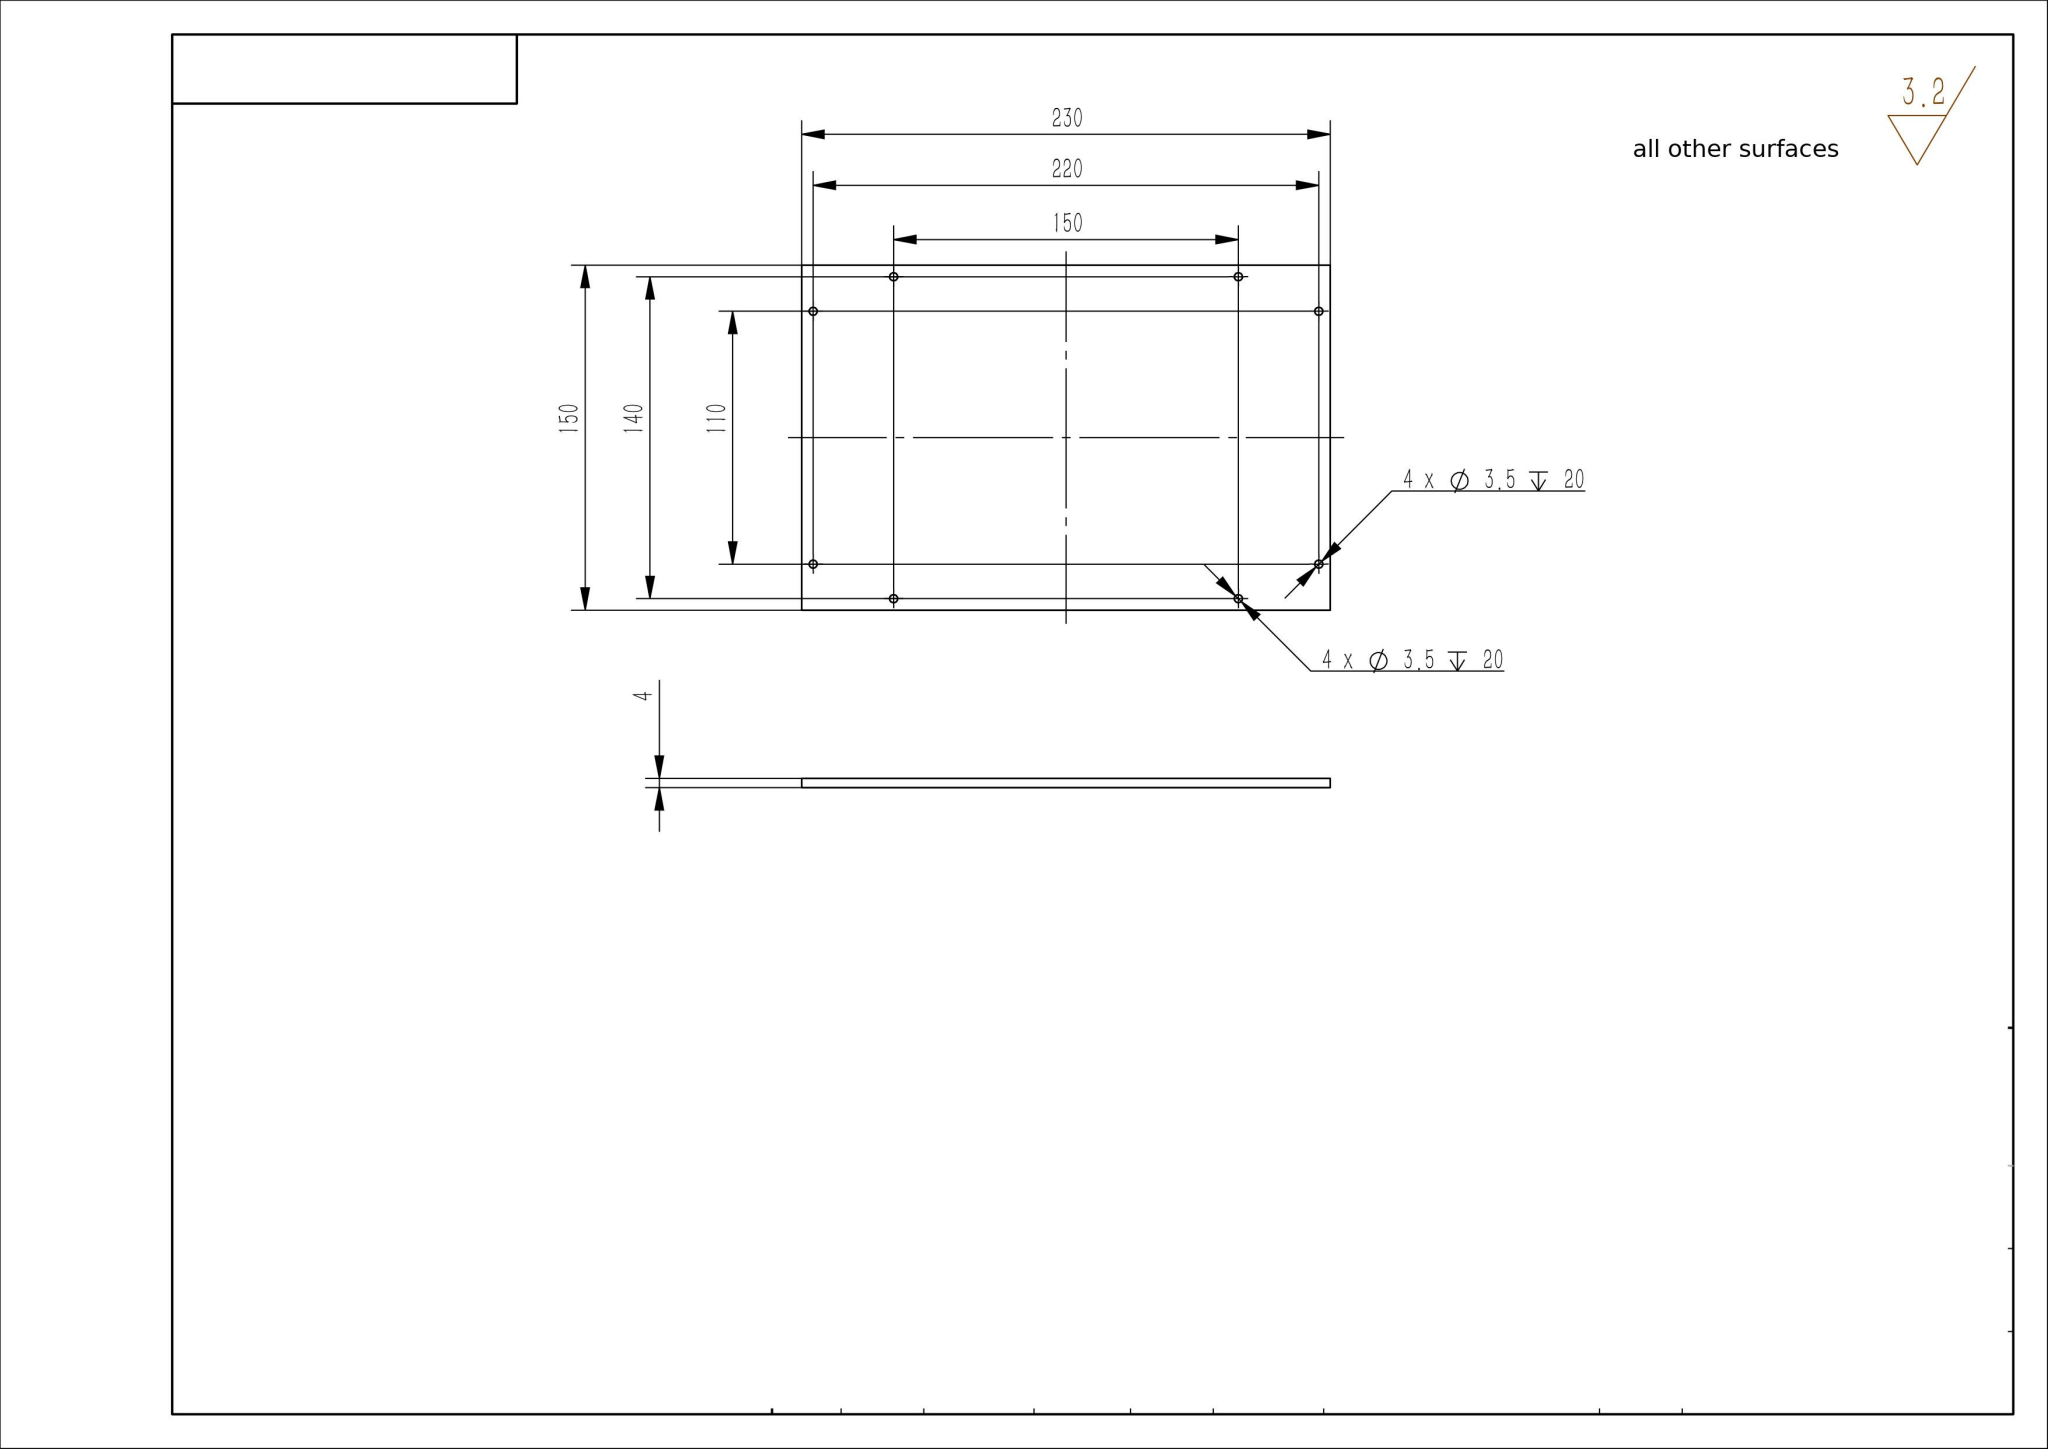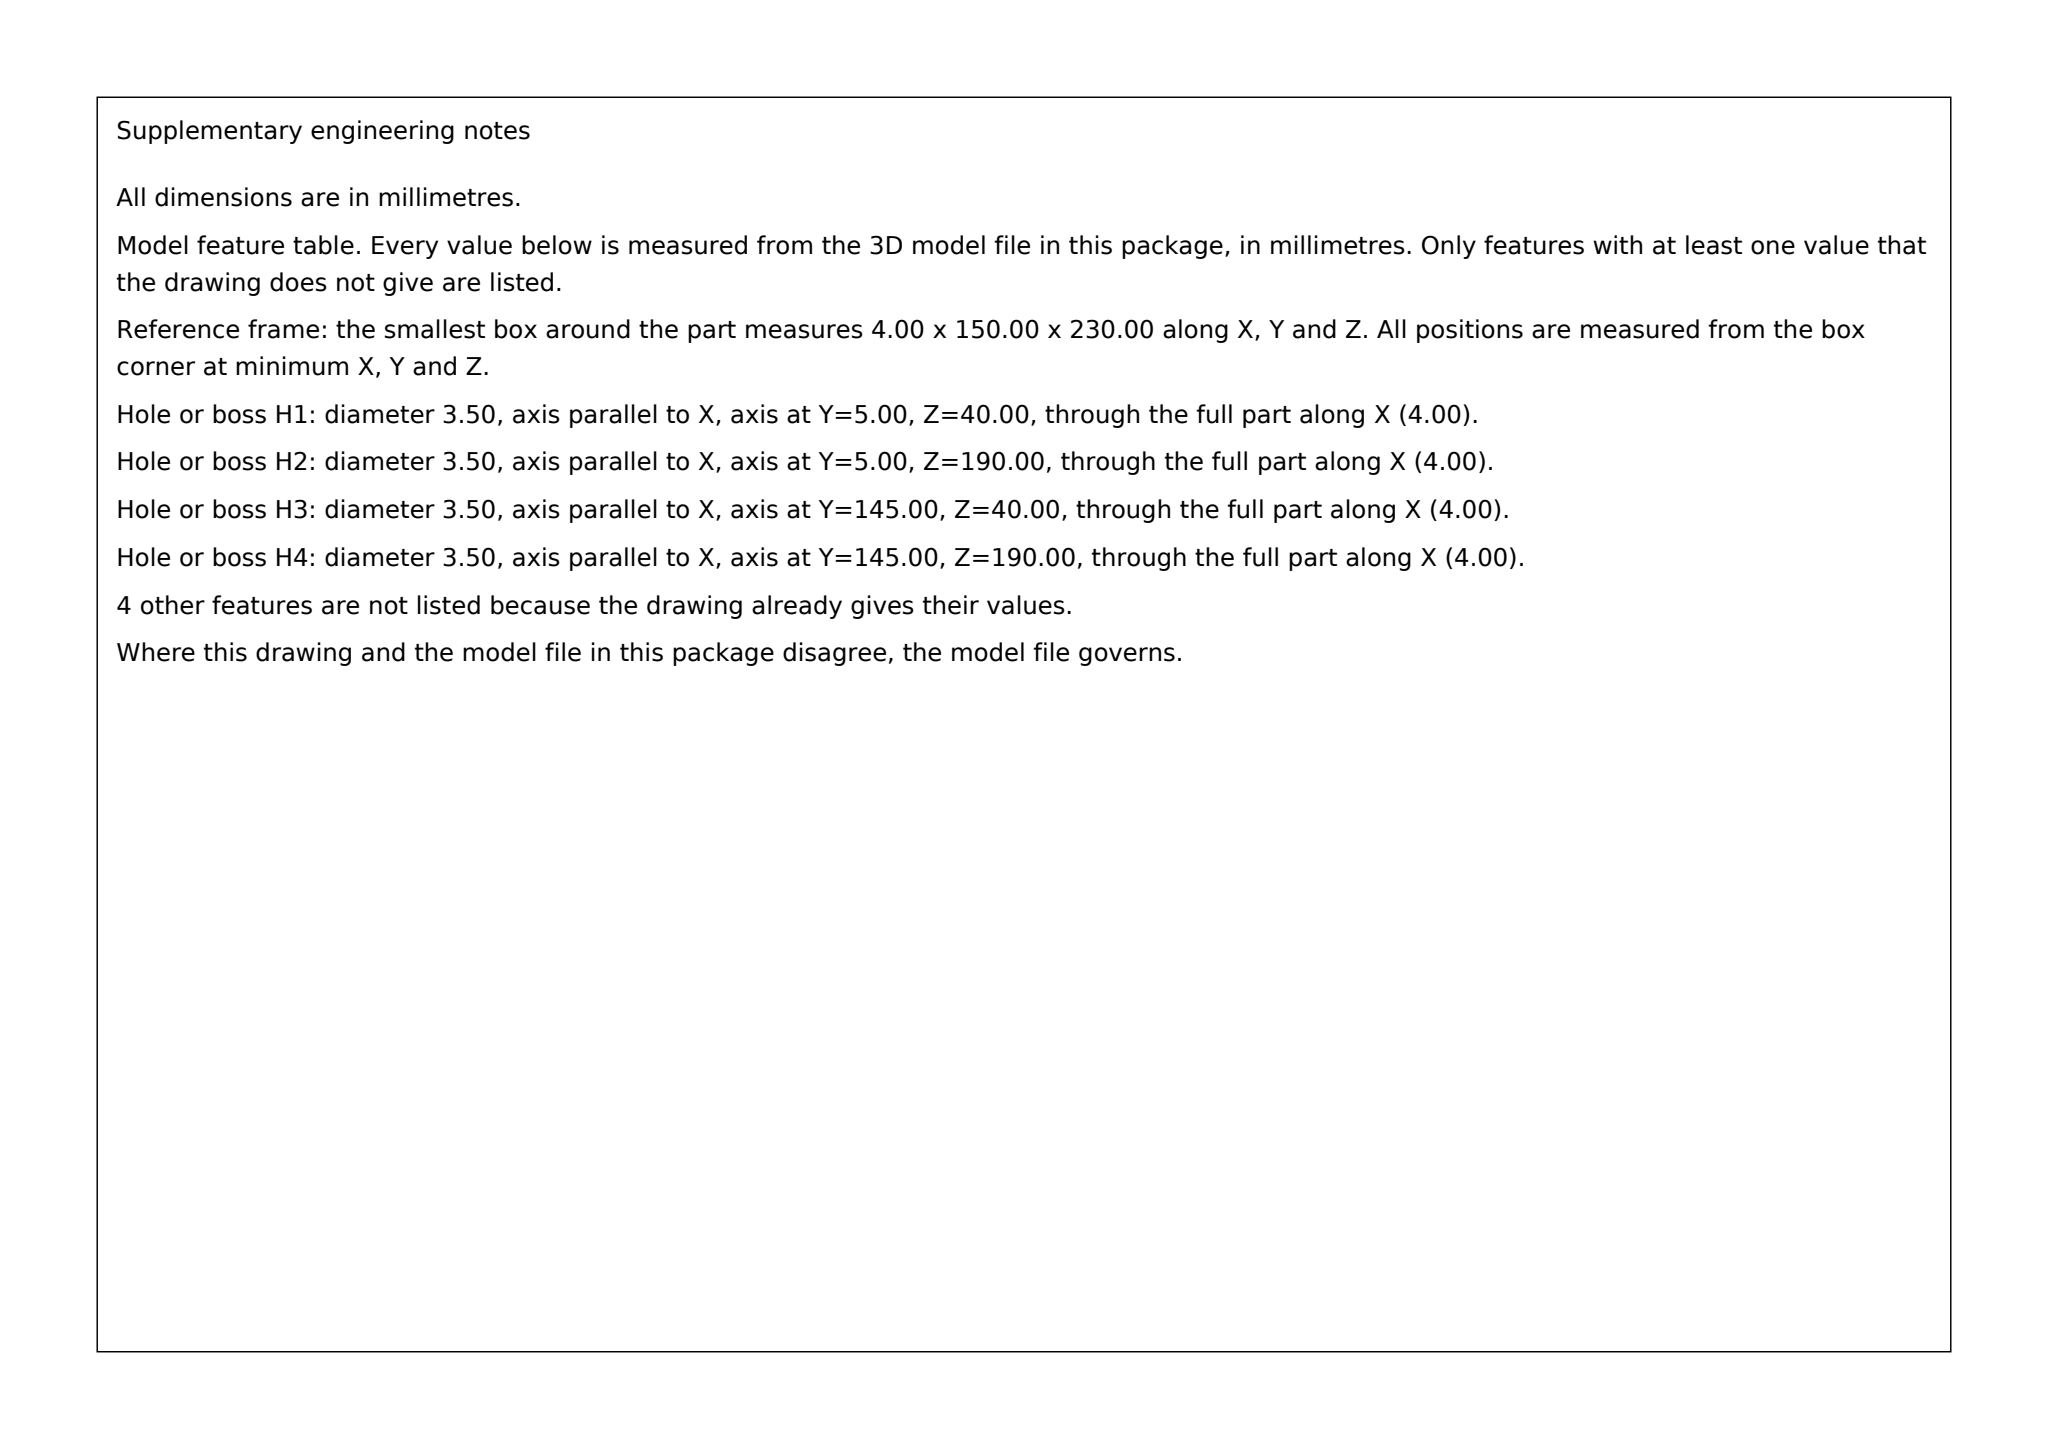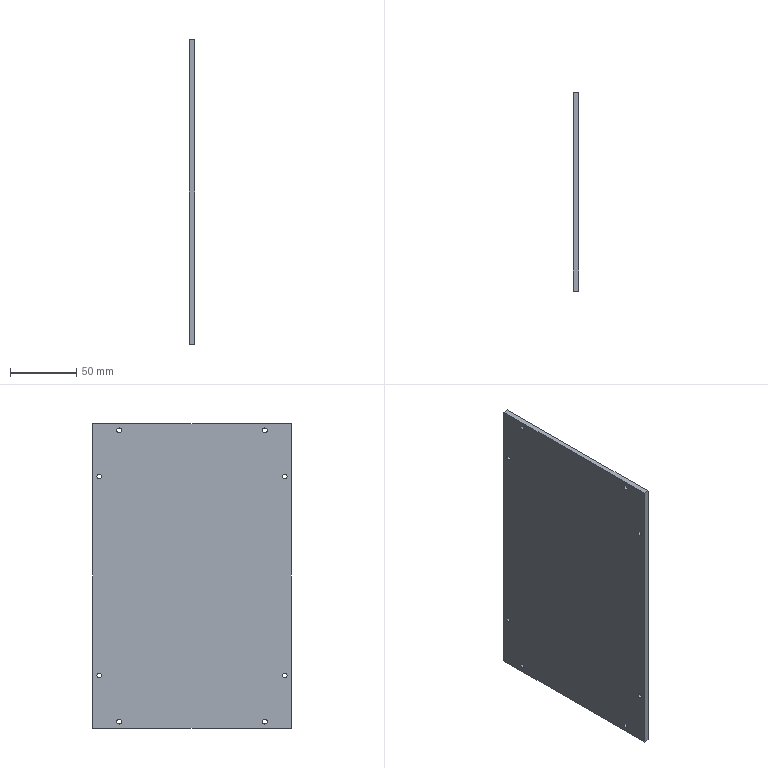Part | SolidWorks | mm | 1 solid | 22 faces | box 4 x 150 x 230 mm | volume 137692 mm3 | cylinder 16 | plane 6 | commonest cylinder face diameters 3.5 x16
build123d program:
from build123d import *

# Parameters (mm, degrees)
SKETCH1_W                           = 230
SKETCH1_H                           = 150
BOSS_EXTRUDE1_DEPTH                 = 4
F_3_5_3_5_DIAMETER_HOLE1_AT_2_COUNT = 2
F_3_5_3_5_DIAMETER_HOLE1_AT_2_PITCH = 110
F_3_5_3_5_DIAMETER_HOLE1_AT_3_COUNT = 2
F_3_5_3_5_DIAMETER_HOLE1_AT_3_PITCH = 38.079
F_3_5_3_5_DIAMETER_HOLE1_AT_4_COUNT = 2
F_3_5_3_5_DIAMETER_HOLE1_AT_4_PITCH = 129.808


with BuildPart() as part:
    # Sketch1 → Boss-Extrude1 (new body)
    with BuildSketch(Plane(origin=(0, 0, 0), x_dir=(0, 0, -1), z_dir=(1, 0, 0))):
        Rectangle(SKETCH1_W, SKETCH1_H)
    extrude(amount=BOSS_EXTRUDE1_DEPTH)

    # Sketch2 → 3.5 _3.5_ Diameter Hole1 (revolve, cut)
    with BuildSketch(Plane(origin=(4, 55, 110), x_dir=(0, 0, -1), z_dir=(0, 1, 0))):
        Polygon((0, 0), (0, 21.052), (1.75, 20), (1.75, 0), align=None)
    f_3_5_3_5_diameter_hole1 = revolve(axis=Axis((10.35, 55, 110), (-1, 0, 0)), mode=Mode.SUBTRACT)

    # 3.5 _3.5_ Diameter Hole1 at 2: 3.5 _3.5_ Diameter Hole1 ×2
    with Locations(*[(0, -i * F_3_5_3_5_DIAMETER_HOLE1_AT_2_PITCH, 0) for i in range(1, F_3_5_3_5_DIAMETER_HOLE1_AT_2_COUNT)]):
        add(f_3_5_3_5_diameter_hole1, mode=Mode.SUBTRACT)

    # 3.5 _3.5_ Diameter Hole1 at 3: 3.5 _3.5_ Diameter Hole1 ×2
    with Locations(*[Vector(0, 0.3939, -0.9191) * (i * F_3_5_3_5_DIAMETER_HOLE1_AT_3_PITCH) for i in range(1, F_3_5_3_5_DIAMETER_HOLE1_AT_3_COUNT)]):
        add(f_3_5_3_5_diameter_hole1, mode=Mode.SUBTRACT)

    # 3.5 _3.5_ Diameter Hole1 at 4: 3.5 _3.5_ Diameter Hole1 ×2
    with Locations(*[Vector(0, -0.963, -0.2696) * (i * F_3_5_3_5_DIAMETER_HOLE1_AT_4_PITCH) for i in range(1, F_3_5_3_5_DIAMETER_HOLE1_AT_4_COUNT)]):
        add(f_3_5_3_5_diameter_hole1, mode=Mode.SUBTRACT)

    # Mirror1: 3.5 _3.5_ Diameter Hole1 across plane
    add(f_3_5_3_5_diameter_hole1.mirror(Plane.XY), mode=Mode.SUBTRACT)

    # Mirror1 copy 1 sketch → Mirror1 copy 1 (revolve, cut)
    with BuildSketch(Plane(origin=(4, -55, -110), x_dir=(0, 0, 1), z_dir=(0, 1, 0))):
        Polygon((0, 0), (0, -21.052), (1.75, -20), (1.75, 0), align=None)
    revolve(axis=Axis((10.35, -55, -110), (1, 0, 0)), mode=Mode.SUBTRACT)

    # Mirror1 copy 2 sketch → Mirror1 copy 2 (revolve, cut)
    with BuildSketch(Plane(origin=(4, 70, -75), x_dir=(0, 0, 1), z_dir=(0, 1, 0))):
        Polygon((0, 0), (0, -21.052), (1.75, -20), (1.75, 0), align=None)
    revolve(axis=Axis((10.35, 70, -75), (1, 0, 0)), mode=Mode.SUBTRACT)

    # Mirror1 copy 3 sketch → Mirror1 copy 3 (revolve, cut)
    with BuildSketch(Plane(origin=(4, -70, -75), x_dir=(0, 0, 1), z_dir=(0, 1, 0))):
        Polygon((0, 0), (0, -21.052), (1.75, -20), (1.75, 0), align=None)
    revolve(axis=Axis((10.35, -70, -75), (1, 0, 0)), mode=Mode.SUBTRACT)


solid = part.part
STEP:
#1=CARTESIAN_POINT('',(0.,55.,-111.75));
#2=VERTEX_POINT('',#1);
#3=CARTESIAN_POINT('',(0.,55.,-108.25));
#4=VERTEX_POINT('',#3);
#5=CARTESIAN_POINT('',(0.,55.,-110.));
#6=DIRECTION('',(-1.,0.,0.));
#7=DIRECTION('',(0.,0.,1.));
#8=AXIS2_PLACEMENT_3D('',#5,#6,#7);
#9=CIRCLE('',#8,1.75);
#10=EDGE_CURVE('',#2,#4,#9,.T.);
#11=ORIENTED_EDGE('',*,*,#10,.T.);
#12=CARTESIAN_POINT('',(4.,55.,-108.25));
#13=VERTEX_POINT('',#12);
#14=CARTESIAN_POINT('',(4.,55.,-108.25));
#15=DIRECTION('',(1.,0.,0.));
#16=VECTOR('',#15,1000.);
#17=LINE('',#14,#16);
#18=EDGE_CURVE('',#4,#13,#17,.T.);
#19=ORIENTED_EDGE('',*,*,#18,.T.);
#20=CARTESIAN_POINT('',(4.,55.,-111.75));
#21=VERTEX_POINT('',#20);
#22=CARTESIAN_POINT('',(4.,55.,-110.));
#23=DIRECTION('',(1.,0.,0.));
#24=DIRECTION('',(0.,0.,-1.));
#25=AXIS2_PLACEMENT_3D('',#22,#23,#24);
#26=CIRCLE('',#25,1.75);
#27=EDGE_CURVE('',#13,#21,#26,.T.);
#28=ORIENTED_EDGE('',*,*,#27,.T.);
#29=CARTESIAN_POINT('',(4.,55.,-111.75));
#30=DIRECTION('',(1.,0.,0.));
#31=VECTOR('',#30,1000.);
#32=LINE('',#29,#31);
#33=EDGE_CURVE('',#2,#21,#32,.T.);
#34=ORIENTED_EDGE('',*,*,#33,.F.);
#35=EDGE_LOOP('',(#11,#19,#28,#34));
#36=FACE_OUTER_BOUND('',#35,.T.);
#37=CARTESIAN_POINT('',(4.,55.,-110.));
#38=DIRECTION('',(1.,0.,0.));
#39=DIRECTION('',(0.,0.,-1.));
#40=AXIS2_PLACEMENT_3D('',#37,#38,#39);
#41=CYLINDRICAL_SURFACE('',#40,1.75);
#42=ADVANCED_FACE('',(#36),#41,.F.);
#43=CARTESIAN_POINT('',(0.,-55.,-111.75));
#44=VERTEX_POINT('',#43);
#45=CARTESIAN_POINT('',(0.,-55.,-108.25));
#46=VERTEX_POINT('',#45);
#47=CARTESIAN_POINT('',(0.,-55.,-110.));
#48=DIRECTION('',(-1.,0.,0.));
#49=DIRECTION('',(0.,0.,1.));
#50=AXIS2_PLACEMENT_3D('',#47,#48,#49);
#51=CIRCLE('',#50,1.75);
#52=EDGE_CURVE('',#44,#46,#51,.T.);
#53=ORIENTED_EDGE('',*,*,#52,.T.);
#54=CARTESIAN_POINT('',(4.,-55.,-108.25));
#55=VERTEX_POINT('',#54);
#56=CARTESIAN_POINT('',(4.,-55.,-108.25));
#57=DIRECTION('',(1.,0.,0.));
#58=VECTOR('',#57,1000.);
#59=LINE('',#56,#58);
#60=EDGE_CURVE('',#46,#55,#59,.T.);
#61=ORIENTED_EDGE('',*,*,#60,.T.);
#62=CARTESIAN_POINT('',(4.,-55.,-111.75));
#63=VERTEX_POINT('',#62);
#64=CARTESIAN_POINT('',(4.,-55.,-110.));
#65=DIRECTION('',(1.,0.,0.));
#66=DIRECTION('',(0.,0.,-1.));
#67=AXIS2_PLACEMENT_3D('',#64,#65,#66);
#68=CIRCLE('',#67,1.75);
#69=EDGE_CURVE('',#55,#63,#68,.T.);
#70=ORIENTED_EDGE('',*,*,#69,.T.);
#71=CARTESIAN_POINT('',(4.,-55.,-111.75));
#72=DIRECTION('',(1.,0.,0.));
#73=VECTOR('',#72,1000.);
#74=LINE('',#71,#73);
#75=EDGE_CURVE('',#44,#63,#74,.T.);
#76=ORIENTED_EDGE('',*,*,#75,.F.);
#77=EDGE_LOOP('',(#53,#61,#70,#76));
#78=FACE_OUTER_BOUND('',#77,.T.);
#79=CARTESIAN_POINT('',(4.,-55.,-110.));
#80=DIRECTION('',(1.,0.,0.));
#81=DIRECTION('',(0.,0.,-1.));
#82=AXIS2_PLACEMENT_3D('',#79,#80,#81);
#83=CYLINDRICAL_SURFACE('',#82,1.75);
#84=ADVANCED_FACE('',(#78),#83,.F.);
#85=CARTESIAN_POINT('',(0.,70.,-76.75));
#86=VERTEX_POINT('',#85);
#87=CARTESIAN_POINT('',(0.,70.,-73.25));
#88=VERTEX_POINT('',#87);
#89=CARTESIAN_POINT('',(0.,70.,-75.));
#90=DIRECTION('',(-1.,0.,0.));
#91=DIRECTION('',(0.,0.,1.));
#92=AXIS2_PLACEMENT_3D('',#89,#90,#91);
#93=CIRCLE('',#92,1.75);
#94=EDGE_CURVE('',#86,#88,#93,.T.);
#95=ORIENTED_EDGE('',*,*,#94,.T.);
#96=CARTESIAN_POINT('',(4.,70.,-73.25));
#97=VERTEX_POINT('',#96);
#98=CARTESIAN_POINT('',(4.,70.,-73.25));
#99=DIRECTION('',(1.,0.,0.));
#100=VECTOR('',#99,1000.);
#101=LINE('',#98,#100);
#102=EDGE_CURVE('',#88,#97,#101,.T.);
#103=ORIENTED_EDGE('',*,*,#102,.T.);
#104=CARTESIAN_POINT('',(4.,70.,-76.75));
#105=VERTEX_POINT('',#104);
#106=CARTESIAN_POINT('',(4.,70.,-75.));
#107=DIRECTION('',(1.,0.,0.));
#108=DIRECTION('',(0.,0.,-1.));
#109=AXIS2_PLACEMENT_3D('',#106,#107,#108);
#110=CIRCLE('',#109,1.75);
#111=EDGE_CURVE('',#97,#105,#110,.T.);
#112=ORIENTED_EDGE('',*,*,#111,.T.);
#113=CARTESIAN_POINT('',(4.,70.,-76.75));
#114=DIRECTION('',(1.,0.,0.));
#115=VECTOR('',#114,1000.);
#116=LINE('',#113,#115);
#117=EDGE_CURVE('',#86,#105,#116,.T.);
#118=ORIENTED_EDGE('',*,*,#117,.F.);
#119=EDGE_LOOP('',(#95,#103,#112,#118));
#120=FACE_OUTER_BOUND('',#119,.T.);
#121=CARTESIAN_POINT('',(4.,70.,-75.));
#122=DIRECTION('',(1.,0.,0.));
#123=DIRECTION('',(0.,0.,-1.));
#124=AXIS2_PLACEMENT_3D('',#121,#122,#123);
#125=CYLINDRICAL_SURFACE('',#124,1.75);
#126=ADVANCED_FACE('',(#120),#125,.F.);
#127=CARTESIAN_POINT('',(0.,-70.,-76.75));
#128=VERTEX_POINT('',#127);
#129=CARTESIAN_POINT('',(0.,-70.,-73.25));
#130=VERTEX_POINT('',#129);
#131=CARTESIAN_POINT('',(0.,-70.,-75.));
#132=DIRECTION('',(-1.,0.,0.));
#133=DIRECTION('',(0.,0.,1.));
#134=AXIS2_PLACEMENT_3D('',#131,#132,#133);
#135=CIRCLE('',#134,1.75);
#136=EDGE_CURVE('',#128,#130,#135,.T.);
#137=ORIENTED_EDGE('',*,*,#136,.T.);
#138=CARTESIAN_POINT('',(4.,-70.,-73.25));
#139=VERTEX_POINT('',#138);
#140=CARTESIAN_POINT('',(4.,-70.,-73.25));
#141=DIRECTION('',(1.,0.,0.));
#142=VECTOR('',#141,1000.);
#143=LINE('',#140,#142);
#144=EDGE_CURVE('',#130,#139,#143,.T.);
#145=ORIENTED_EDGE('',*,*,#144,.T.);
#146=CARTESIAN_POINT('',(4.,-70.,-76.75));
#147=VERTEX_POINT('',#146);
#148=CARTESIAN_POINT('',(4.,-70.,-75.));
#149=DIRECTION('',(1.,0.,0.));
#150=DIRECTION('',(0.,0.,-1.));
#151=AXIS2_PLACEMENT_3D('',#148,#149,#150);
#152=CIRCLE('',#151,1.75);
#153=EDGE_CURVE('',#139,#147,#152,.T.);
#154=ORIENTED_EDGE('',*,*,#153,.T.);
#155=CARTESIAN_POINT('',(4.,-70.,-76.75));
#156=DIRECTION('',(1.,0.,0.));
#157=VECTOR('',#156,1000.);
#158=LINE('',#155,#157);
#159=EDGE_CURVE('',#128,#147,#158,.T.);
#160=ORIENTED_EDGE('',*,*,#159,.F.);
#161=EDGE_LOOP('',(#137,#145,#154,#160));
#162=FACE_OUTER_BOUND('',#161,.T.);
#163=CARTESIAN_POINT('',(4.,-70.,-75.));
#164=DIRECTION('',(1.,0.,0.));
#165=DIRECTION('',(0.,0.,-1.));
#166=AXIS2_PLACEMENT_3D('',#163,#164,#165);
#167=CYLINDRICAL_SURFACE('',#166,1.75);
#168=ADVANCED_FACE('',(#162),#167,.F.);
#169=CARTESIAN_POINT('',(0.,55.,108.25));
#170=VERTEX_POINT('',#169);
#171=CARTESIAN_POINT('',(0.,55.,111.75));
#172=VERTEX_POINT('',#171);
#173=CARTESIAN_POINT('',(0.,55.,110.));
#174=DIRECTION('',(-1.,0.,0.));
#175=DIRECTION('',(0.,0.,1.));
#176=AXIS2_PLACEMENT_3D('',#173,#174,#175);
#177=CIRCLE('',#176,1.75);
#178=EDGE_CURVE('',#170,#172,#177,.T.);
#179=ORIENTED_EDGE('',*,*,#178,.T.);
#180=CARTESIAN_POINT('',(4.,55.,111.75));
#181=VERTEX_POINT('',#180);
#182=CARTESIAN_POINT('',(4.,55.,111.75));
#183=DIRECTION('',(1.,0.,0.));
#184=VECTOR('',#183,1000.);
#185=LINE('',#182,#184);
#186=EDGE_CURVE('',#172,#181,#185,.T.);
#187=ORIENTED_EDGE('',*,*,#186,.T.);
#188=CARTESIAN_POINT('',(4.,55.,108.25));
#189=VERTEX_POINT('',#188);
#190=CARTESIAN_POINT('',(4.,55.,110.));
#191=DIRECTION('',(1.,0.,0.));
#192=DIRECTION('',(0.,0.,-1.));
#193=AXIS2_PLACEMENT_3D('',#190,#191,#192);
#194=CIRCLE('',#193,1.75);
#195=EDGE_CURVE('',#181,#189,#194,.T.);
#196=ORIENTED_EDGE('',*,*,#195,.T.);
#197=CARTESIAN_POINT('',(4.,55.,108.25));
#198=DIRECTION('',(1.,0.,0.));
#199=VECTOR('',#198,1000.);
#200=LINE('',#197,#199);
#201=EDGE_CURVE('',#170,#189,#200,.T.);
#202=ORIENTED_EDGE('',*,*,#201,.F.);
#203=EDGE_LOOP('',(#179,#187,#196,#202));
#204=FACE_OUTER_BOUND('',#203,.T.);
#205=CARTESIAN_POINT('',(4.,55.,110.));
#206=DIRECTION('',(1.,0.,0.));
#207=DIRECTION('',(0.,0.,-1.));
#208=AXIS2_PLACEMENT_3D('',#205,#206,#207);
#209=CYLINDRICAL_SURFACE('',#208,1.75);
#210=ADVANCED_FACE('',(#204),#209,.F.);
#211=CARTESIAN_POINT('',(0.,-55.,108.25));
#212=VERTEX_POINT('',#211);
#213=CARTESIAN_POINT('',(0.,-55.,111.75));
#214=VERTEX_POINT('',#213);
#215=CARTESIAN_POINT('',(0.,-55.,110.));
#216=DIRECTION('',(-1.,0.,0.));
#217=DIRECTION('',(0.,0.,1.));
#218=AXIS2_PLACEMENT_3D('',#215,#216,#217);
#219=CIRCLE('',#218,1.75);
#220=EDGE_CURVE('',#212,#214,#219,.T.);
#221=ORIENTED_EDGE('',*,*,#220,.T.);
#222=CARTESIAN_POINT('',(4.,-55.,111.75));
#223=VERTEX_POINT('',#222);
#224=CARTESIAN_POINT('',(4.,-55.,111.75));
#225=DIRECTION('',(1.,0.,0.));
#226=VECTOR('',#225,1000.);
#227=LINE('',#224,#226);
#228=EDGE_CURVE('',#214,#223,#227,.T.);
#229=ORIENTED_EDGE('',*,*,#228,.T.);
#230=CARTESIAN_POINT('',(4.,-55.,108.25));
#231=VERTEX_POINT('',#230);
#232=CARTESIAN_POINT('',(4.,-55.,110.));
#233=DIRECTION('',(1.,0.,0.));
#234=DIRECTION('',(0.,0.,-1.));
#235=AXIS2_PLACEMENT_3D('',#232,#233,#234);
#236=CIRCLE('',#235,1.75);
#237=EDGE_CURVE('',#223,#231,#236,.T.);
#238=ORIENTED_EDGE('',*,*,#237,.T.);
#239=CARTESIAN_POINT('',(4.,-55.,108.25));
#240=DIRECTION('',(1.,0.,0.));
#241=VECTOR('',#240,1000.);
#242=LINE('',#239,#241);
#243=EDGE_CURVE('',#212,#231,#242,.T.);
#244=ORIENTED_EDGE('',*,*,#243,.F.);
#245=EDGE_LOOP('',(#221,#229,#238,#244));
#246=FACE_OUTER_BOUND('',#245,.T.);
#247=CARTESIAN_POINT('',(4.,-55.,110.));
#248=DIRECTION('',(1.,0.,0.));
#249=DIRECTION('',(0.,0.,-1.));
#250=AXIS2_PLACEMENT_3D('',#247,#248,#249);
#251=CYLINDRICAL_SURFACE('',#250,1.75);
#252=ADVANCED_FACE('',(#246),#251,.F.);
#253=CARTESIAN_POINT('',(0.,70.,73.25));
#254=VERTEX_POINT('',#253);
#255=CARTESIAN_POINT('',(0.,70.,76.75));
#256=VERTEX_POINT('',#255);
#257=CARTESIAN_POINT('',(0.,70.,75.));
#258=DIRECTION('',(-1.,0.,0.));
#259=DIRECTION('',(0.,0.,1.));
#260=AXIS2_PLACEMENT_3D('',#257,#258,#259);
#261=CIRCLE('',#260,1.75);
#262=EDGE_CURVE('',#254,#256,#261,.T.);
#263=ORIENTED_EDGE('',*,*,#262,.T.);
#264=CARTESIAN_POINT('',(4.,70.,76.75));
#265=VERTEX_POINT('',#264);
#266=CARTESIAN_POINT('',(4.,70.,76.75));
#267=DIRECTION('',(1.,0.,0.));
#268=VECTOR('',#267,1000.);
#269=LINE('',#266,#268);
#270=EDGE_CURVE('',#256,#265,#269,.T.);
#271=ORIENTED_EDGE('',*,*,#270,.T.);
#272=CARTESIAN_POINT('',(4.,70.,73.25));
#273=VERTEX_POINT('',#272);
#274=CARTESIAN_POINT('',(4.,70.,75.));
#275=DIRECTION('',(1.,0.,0.));
#276=DIRECTION('',(0.,0.,-1.));
#277=AXIS2_PLACEMENT_3D('',#274,#275,#276);
#278=CIRCLE('',#277,1.75);
#279=EDGE_CURVE('',#265,#273,#278,.T.);
#280=ORIENTED_EDGE('',*,*,#279,.T.);
#281=CARTESIAN_POINT('',(4.,70.,73.25));
#282=DIRECTION('',(1.,0.,0.));
#283=VECTOR('',#282,1000.);
#284=LINE('',#281,#283);
#285=EDGE_CURVE('',#254,#273,#284,.T.);
#286=ORIENTED_EDGE('',*,*,#285,.F.);
#287=EDGE_LOOP('',(#263,#271,#280,#286));
#288=FACE_OUTER_BOUND('',#287,.T.);
#289=CARTESIAN_POINT('',(4.,70.,75.));
#290=DIRECTION('',(1.,0.,0.));
#291=DIRECTION('',(0.,0.,-1.));
#292=AXIS2_PLACEMENT_3D('',#289,#290,#291);
#293=CYLINDRICAL_SURFACE('',#292,1.75);
#294=ADVANCED_FACE('',(#288),#293,.F.);
#295=CARTESIAN_POINT('',(0.,-70.,73.25));
#296=VERTEX_POINT('',#295);
#297=CARTESIAN_POINT('',(0.,-70.,76.75));
#298=VERTEX_POINT('',#297);
#299=CARTESIAN_POINT('',(0.,-70.,75.));
#300=DIRECTION('',(-1.,0.,0.));
#301=DIRECTION('',(0.,0.,1.));
#302=AXIS2_PLACEMENT_3D('',#299,#300,#301);
#303=CIRCLE('',#302,1.75);
#304=EDGE_CURVE('',#296,#298,#303,.T.);
#305=ORIENTED_EDGE('',*,*,#304,.T.);
#306=CARTESIAN_POINT('',(4.,-70.,76.75));
#307=VERTEX_POINT('',#306);
#308=CARTESIAN_POINT('',(4.,-70.,76.75));
#309=DIRECTION('',(1.,0.,0.));
#310=VECTOR('',#309,1000.);
#311=LINE('',#308,#310);
#312=EDGE_CURVE('',#298,#307,#311,.T.);
#313=ORIENTED_EDGE('',*,*,#312,.T.);
#314=CARTESIAN_POINT('',(4.,-70.,73.25));
#315=VERTEX_POINT('',#314);
#316=CARTESIAN_POINT('',(4.,-70.,75.));
#317=DIRECTION('',(1.,0.,0.));
#318=DIRECTION('',(0.,0.,-1.));
#319=AXIS2_PLACEMENT_3D('',#316,#317,#318);
#320=CIRCLE('',#319,1.75);
#321=EDGE_CURVE('',#307,#315,#320,.T.);
#322=ORIENTED_EDGE('',*,*,#321,.T.);
#323=CARTESIAN_POINT('',(4.,-70.,73.25));
#324=DIRECTION('',(1.,0.,0.));
#325=VECTOR('',#324,1000.);
#326=LINE('',#323,#325);
#327=EDGE_CURVE('',#296,#315,#326,.T.);
#328=ORIENTED_EDGE('',*,*,#327,.F.);
#329=EDGE_LOOP('',(#305,#313,#322,#328));
#330=FACE_OUTER_BOUND('',#329,.T.);
#331=CARTESIAN_POINT('',(4.,-70.,75.));
#332=DIRECTION('',(1.,0.,0.));
#333=DIRECTION('',(0.,0.,-1.));
#334=AXIS2_PLACEMENT_3D('',#331,#332,#333);
#335=CYLINDRICAL_SURFACE('',#334,1.75);
#336=ADVANCED_FACE('',(#330),#335,.F.);
#337=CARTESIAN_POINT('',(0.,-75.,-115.));
#338=VERTEX_POINT('',#337);
#339=CARTESIAN_POINT('',(0.,75.,-115.));
#340=VERTEX_POINT('',#339);
#341=CARTESIAN_POINT('',(0.,-75.,-115.));
#342=DIRECTION('',(0.,1.,0.));
#343=VECTOR('',#342,1000.);
#344=LINE('',#341,#343);
#345=EDGE_CURVE('',#338,#340,#344,.T.);
#346=ORIENTED_EDGE('',*,*,#345,.T.);
#347=CARTESIAN_POINT('',(4.,75.,-115.));
#348=VERTEX_POINT('',#347);
#349=CARTESIAN_POINT('',(4.,75.,-115.));
#350=DIRECTION('',(-1.,0.,0.));
#351=VECTOR('',#350,1000.);
#352=LINE('',#349,#351);
#353=EDGE_CURVE('',#348,#340,#352,.T.);
#354=ORIENTED_EDGE('',*,*,#353,.F.);
#355=CARTESIAN_POINT('',(4.,-75.,-115.));
#356=VERTEX_POINT('',#355);
#357=CARTESIAN_POINT('',(4.,-75.,-115.));
#358=DIRECTION('',(0.,1.,0.));
#359=VECTOR('',#358,1000.);
#360=LINE('',#357,#359);
#361=EDGE_CURVE('',#356,#348,#360,.T.);
#362=ORIENTED_EDGE('',*,*,#361,.F.);
#363=CARTESIAN_POINT('',(4.,-75.,-115.));
#364=DIRECTION('',(-1.,0.,0.));
#365=VECTOR('',#364,1000.);
#366=LINE('',#363,#365);
#367=EDGE_CURVE('',#356,#338,#366,.T.);
#368=ORIENTED_EDGE('',*,*,#367,.T.);
#369=EDGE_LOOP('',(#346,#354,#362,#368));
#370=FACE_OUTER_BOUND('',#369,.T.);
#371=CARTESIAN_POINT('',(4.,-75.,-115.));
#372=DIRECTION('',(0.,0.,1.));
#373=DIRECTION('',(1.,0.,0.));
#374=AXIS2_PLACEMENT_3D('',#371,#372,#373);
#375=PLANE('',#374);
#376=ADVANCED_FACE('',(#370),#375,.F.);
#377=CARTESIAN_POINT('',(0.,75.,115.));
#378=VERTEX_POINT('',#377);
#379=CARTESIAN_POINT('',(0.,75.,115.));
#380=DIRECTION('',(0.,0.,1.));
#381=VECTOR('',#380,1000.);
#382=LINE('',#379,#381);
#383=EDGE_CURVE('',#340,#378,#382,.T.);
#384=ORIENTED_EDGE('',*,*,#383,.T.);
#385=CARTESIAN_POINT('',(4.,75.,115.));
#386=VERTEX_POINT('',#385);
#387=CARTESIAN_POINT('',(4.,75.,115.));
#388=DIRECTION('',(-1.,0.,0.));
#389=VECTOR('',#388,1000.);
#390=LINE('',#387,#389);
#391=EDGE_CURVE('',#386,#378,#390,.T.);
#392=ORIENTED_EDGE('',*,*,#391,.F.);
#393=CARTESIAN_POINT('',(4.,75.,115.));
#394=DIRECTION('',(0.,0.,1.));
#395=VECTOR('',#394,1000.);
#396=LINE('',#393,#395);
#397=EDGE_CURVE('',#348,#386,#396,.T.);
#398=ORIENTED_EDGE('',*,*,#397,.F.);
#399=ORIENTED_EDGE('',*,*,#353,.T.);
#400=EDGE_LOOP('',(#384,#392,#398,#399));
#401=FACE_OUTER_BOUND('',#400,.T.);
#402=CARTESIAN_POINT('',(4.,75.,115.));
#403=DIRECTION('',(0.,-1.,0.));
#404=DIRECTION('',(0.,0.,-1.));
#405=AXIS2_PLACEMENT_3D('',#402,#403,#404);
#406=PLANE('',#405);
#407=ADVANCED_FACE('',(#401),#406,.F.);
#408=CARTESIAN_POINT('',(0.,-75.,115.));
#409=VERTEX_POINT('',#408);
#410=CARTESIAN_POINT('',(0.,-75.,115.));
#411=DIRECTION('',(0.,-1.,0.));
#412=VECTOR('',#411,1000.);
#413=LINE('',#410,#412);
#414=EDGE_CURVE('',#378,#409,#413,.T.);
#415=ORIENTED_EDGE('',*,*,#414,.T.);
#416=CARTESIAN_POINT('',(4.,-75.,115.));
#417=VERTEX_POINT('',#416);
#418=CARTESIAN_POINT('',(4.,-75.,115.));
#419=DIRECTION('',(-1.,0.,0.));
#420=VECTOR('',#419,1000.);
#421=LINE('',#418,#420);
#422=EDGE_CURVE('',#417,#409,#421,.T.);
#423=ORIENTED_EDGE('',*,*,#422,.F.);
#424=CARTESIAN_POINT('',(4.,-75.,115.));
#425=DIRECTION('',(0.,-1.,0.));
#426=VECTOR('',#425,1000.);
#427=LINE('',#424,#426);
#428=EDGE_CURVE('',#386,#417,#427,.T.);
#429=ORIENTED_EDGE('',*,*,#428,.F.);
#430=ORIENTED_EDGE('',*,*,#391,.T.);
#431=EDGE_LOOP('',(#415,#423,#429,#430));
#432=FACE_OUTER_BOUND('',#431,.T.);
#433=CARTESIAN_POINT('',(4.,-75.,115.));
#434=DIRECTION('',(0.,0.,-1.));
#435=DIRECTION('',(-1.,0.,0.));
#436=AXIS2_PLACEMENT_3D('',#433,#434,#435);
#437=PLANE('',#436);
#438=ADVANCED_FACE('',(#432),#437,.F.);
#439=CARTESIAN_POINT('',(0.,-75.,115.));
#440=DIRECTION('',(0.,0.,-1.));
#441=VECTOR('',#440,1000.);
#442=LINE('',#439,#441);
#443=EDGE_CURVE('',#409,#338,#442,.T.);
#444=ORIENTED_EDGE('',*,*,#443,.T.);
#445=ORIENTED_EDGE('',*,*,#367,.F.);
#446=CARTESIAN_POINT('',(4.,-75.,115.));
#447=DIRECTION('',(0.,0.,-1.));
#448=VECTOR('',#447,1000.);
#449=LINE('',#446,#448);
#450=EDGE_CURVE('',#417,#356,#449,.T.);
#451=ORIENTED_EDGE('',*,*,#450,.F.);
#452=ORIENTED_EDGE('',*,*,#422,.T.);
#453=EDGE_LOOP('',(#444,#445,#451,#452));
#454=FACE_OUTER_BOUND('',#453,.T.);
#455=CARTESIAN_POINT('',(4.,-75.,115.));
#456=DIRECTION('',(0.,1.,0.));
#457=DIRECTION('',(0.,0.,1.));
#458=AXIS2_PLACEMENT_3D('',#455,#456,#457);
#459=PLANE('',#458);
#460=ADVANCED_FACE('',(#454),#459,.F.);
#461=CARTESIAN_POINT('',(4.,55.,-110.));
#462=DIRECTION('',(1.,0.,0.));
#463=DIRECTION('',(0.,0.,-1.));
#464=AXIS2_PLACEMENT_3D('',#461,#462,#463);
#465=CIRCLE('',#464,1.75);
#466=EDGE_CURVE('',#21,#13,#465,.T.);
#467=ORIENTED_EDGE('',*,*,#466,.F.);
#468=ORIENTED_EDGE('',*,*,#27,.F.);
#469=EDGE_LOOP('',(#467,#468));
#470=FACE_BOUND('',#469,.T.);
#471=CARTESIAN_POINT('',(4.,-55.,-110.));
#472=DIRECTION('',(1.,0.,0.));
#473=DIRECTION('',(0.,0.,-1.));
#474=AXIS2_PLACEMENT_3D('',#471,#472,#473);
#475=CIRCLE('',#474,1.75);
#476=EDGE_CURVE('',#63,#55,#475,.T.);
#477=ORIENTED_EDGE('',*,*,#476,.F.);
#478=ORIENTED_EDGE('',*,*,#69,.F.);
#479=EDGE_LOOP('',(#477,#478));
#480=FACE_BOUND('',#479,.T.);
#481=CARTESIAN_POINT('',(4.,70.,-75.));
#482=DIRECTION('',(1.,0.,0.));
#483=DIRECTION('',(0.,0.,-1.));
#484=AXIS2_PLACEMENT_3D('',#481,#482,#483);
#485=CIRCLE('',#484,1.75);
#486=EDGE_CURVE('',#105,#97,#485,.T.);
#487=ORIENTED_EDGE('',*,*,#486,.F.);
#488=ORIENTED_EDGE('',*,*,#111,.F.);
#489=EDGE_LOOP('',(#487,#488));
#490=FACE_BOUND('',#489,.T.);
#491=CARTESIAN_POINT('',(4.,-70.,-75.));
#492=DIRECTION('',(1.,0.,0.));
#493=DIRECTION('',(0.,0.,-1.));
#494=AXIS2_PLACEMENT_3D('',#491,#492,#493);
#495=CIRCLE('',#494,1.75);
#496=EDGE_CURVE('',#147,#139,#495,.T.);
#497=ORIENTED_EDGE('',*,*,#496,.F.);
#498=ORIENTED_EDGE('',*,*,#153,.F.);
#499=EDGE_LOOP('',(#497,#498));
#500=FACE_BOUND('',#499,.T.);
#501=CARTESIAN_POINT('',(4.,55.,110.));
#502=DIRECTION('',(1.,0.,0.));
#503=DIRECTION('',(0.,0.,-1.));
#504=AXIS2_PLACEMENT_3D('',#501,#502,#503);
#505=CIRCLE('',#504,1.75);
#506=EDGE_CURVE('',#189,#181,#505,.T.);
#507=ORIENTED_EDGE('',*,*,#506,.F.);
#508=ORIENTED_EDGE('',*,*,#195,.F.);
#509=EDGE_LOOP('',(#507,#508));
#510=FACE_BOUND('',#509,.T.);
#511=CARTESIAN_POINT('',(4.,-55.,110.));
#512=DIRECTION('',(1.,0.,0.));
#513=DIRECTION('',(0.,0.,-1.));
#514=AXIS2_PLACEMENT_3D('',#511,#512,#513);
#515=CIRCLE('',#514,1.75);
#516=EDGE_CURVE('',#231,#223,#515,.T.);
#517=ORIENTED_EDGE('',*,*,#516,.F.);
#518=ORIENTED_EDGE('',*,*,#237,.F.);
#519=EDGE_LOOP('',(#517,#518));
#520=FACE_BOUND('',#519,.T.);
#521=CARTESIAN_POINT('',(4.,70.,75.));
#522=DIRECTION('',(1.,0.,0.));
#523=DIRECTION('',(0.,0.,-1.));
#524=AXIS2_PLACEMENT_3D('',#521,#522,#523);
#525=CIRCLE('',#524,1.75);
#526=EDGE_CURVE('',#273,#265,#525,.T.);
#527=ORIENTED_EDGE('',*,*,#526,.F.);
#528=ORIENTED_EDGE('',*,*,#279,.F.);
#529=EDGE_LOOP('',(#527,#528));
#530=FACE_BOUND('',#529,.T.);
#531=CARTESIAN_POINT('',(4.,-70.,75.));
#532=DIRECTION('',(1.,0.,0.));
#533=DIRECTION('',(0.,0.,-1.));
#534=AXIS2_PLACEMENT_3D('',#531,#532,#533);
#535=CIRCLE('',#534,1.75);
#536=EDGE_CURVE('',#315,#307,#535,.T.);
#537=ORIENTED_EDGE('',*,*,#536,.F.);
#538=ORIENTED_EDGE('',*,*,#321,.F.);
#539=EDGE_LOOP('',(#537,#538));
#540=FACE_BOUND('',#539,.T.);
#541=ORIENTED_EDGE('',*,*,#361,.T.);
#542=ORIENTED_EDGE('',*,*,#397,.T.);
#543=ORIENTED_EDGE('',*,*,#428,.T.);
#544=ORIENTED_EDGE('',*,*,#450,.T.);
#545=EDGE_LOOP('',(#541,#542,#543,#544));
#546=FACE_OUTER_BOUND('',#545,.T.);
#547=CARTESIAN_POINT('',(4.,0.,0.));
#548=DIRECTION('',(-1.,0.,0.));
#549=DIRECTION('',(0.,0.,1.));
#550=AXIS2_PLACEMENT_3D('',#547,#548,#549);
#551=PLANE('',#550);
#552=ADVANCED_FACE('',(#470,#480,#490,#500,#510,#520,#530,#540,#546),#551,.F.);
#553=ORIENTED_EDGE('',*,*,#10,.F.);
#554=CARTESIAN_POINT('',(0.,55.,-110.));
#555=DIRECTION('',(-1.,0.,0.));
#556=DIRECTION('',(0.,0.,1.));
#557=AXIS2_PLACEMENT_3D('',#554,#555,#556);
#558=CIRCLE('',#557,1.75);
#559=EDGE_CURVE('',#4,#2,#558,.T.);
#560=ORIENTED_EDGE('',*,*,#559,.F.);
#561=EDGE_LOOP('',(#553,#560));
#562=FACE_BOUND('',#561,.T.);
#563=ORIENTED_EDGE('',*,*,#52,.F.);
#564=CARTESIAN_POINT('',(0.,-55.,-110.));
#565=DIRECTION('',(-1.,0.,0.));
#566=DIRECTION('',(0.,0.,1.));
#567=AXIS2_PLACEMENT_3D('',#564,#565,#566);
#568=CIRCLE('',#567,1.75);
#569=EDGE_CURVE('',#46,#44,#568,.T.);
#570=ORIENTED_EDGE('',*,*,#569,.F.);
#571=EDGE_LOOP('',(#563,#570));
#572=FACE_BOUND('',#571,.T.);
#573=ORIENTED_EDGE('',*,*,#94,.F.);
#574=CARTESIAN_POINT('',(0.,70.,-75.));
#575=DIRECTION('',(-1.,0.,0.));
#576=DIRECTION('',(0.,0.,1.));
#577=AXIS2_PLACEMENT_3D('',#574,#575,#576);
#578=CIRCLE('',#577,1.75);
#579=EDGE_CURVE('',#88,#86,#578,.T.);
#580=ORIENTED_EDGE('',*,*,#579,.F.);
#581=EDGE_LOOP('',(#573,#580));
#582=FACE_BOUND('',#581,.T.);
#583=ORIENTED_EDGE('',*,*,#136,.F.);
#584=CARTESIAN_POINT('',(0.,-70.,-75.));
#585=DIRECTION('',(-1.,0.,0.));
#586=DIRECTION('',(0.,0.,1.));
#587=AXIS2_PLACEMENT_3D('',#584,#585,#586);
#588=CIRCLE('',#587,1.75);
#589=EDGE_CURVE('',#130,#128,#588,.T.);
#590=ORIENTED_EDGE('',*,*,#589,.F.);
#591=EDGE_LOOP('',(#583,#590));
#592=FACE_BOUND('',#591,.T.);
#593=ORIENTED_EDGE('',*,*,#178,.F.);
#594=CARTESIAN_POINT('',(0.,55.,110.));
#595=DIRECTION('',(-1.,0.,0.));
#596=DIRECTION('',(0.,0.,1.));
#597=AXIS2_PLACEMENT_3D('',#594,#595,#596);
#598=CIRCLE('',#597,1.75);
#599=EDGE_CURVE('',#172,#170,#598,.T.);
#600=ORIENTED_EDGE('',*,*,#599,.F.);
#601=EDGE_LOOP('',(#593,#600));
#602=FACE_BOUND('',#601,.T.);
#603=ORIENTED_EDGE('',*,*,#220,.F.);
#604=CARTESIAN_POINT('',(0.,-55.,110.));
#605=DIRECTION('',(-1.,0.,0.));
#606=DIRECTION('',(0.,0.,1.));
#607=AXIS2_PLACEMENT_3D('',#604,#605,#606);
#608=CIRCLE('',#607,1.75);
#609=EDGE_CURVE('',#214,#212,#608,.T.);
#610=ORIENTED_EDGE('',*,*,#609,.F.);
#611=EDGE_LOOP('',(#603,#610));
#612=FACE_BOUND('',#611,.T.);
#613=ORIENTED_EDGE('',*,*,#262,.F.);
#614=CARTESIAN_POINT('',(0.,70.,75.));
#615=DIRECTION('',(-1.,0.,0.));
#616=DIRECTION('',(0.,0.,1.));
#617=AXIS2_PLACEMENT_3D('',#614,#615,#616);
#618=CIRCLE('',#617,1.75);
#619=EDGE_CURVE('',#256,#254,#618,.T.);
#620=ORIENTED_EDGE('',*,*,#619,.F.);
#621=EDGE_LOOP('',(#613,#620));
#622=FACE_BOUND('',#621,.T.);
#623=ORIENTED_EDGE('',*,*,#304,.F.);
#624=CARTESIAN_POINT('',(0.,-70.,75.));
#625=DIRECTION('',(-1.,0.,0.));
#626=DIRECTION('',(0.,0.,1.));
#627=AXIS2_PLACEMENT_3D('',#624,#625,#626);
#628=CIRCLE('',#627,1.75);
#629=EDGE_CURVE('',#298,#296,#628,.T.);
#630=ORIENTED_EDGE('',*,*,#629,.F.);
#631=EDGE_LOOP('',(#623,#630));
#632=FACE_BOUND('',#631,.T.);
#633=ORIENTED_EDGE('',*,*,#345,.F.);
#634=ORIENTED_EDGE('',*,*,#443,.F.);
#635=ORIENTED_EDGE('',*,*,#414,.F.);
#636=ORIENTED_EDGE('',*,*,#383,.F.);
#637=EDGE_LOOP('',(#633,#634,#635,#636));
#638=FACE_OUTER_BOUND('',#637,.T.);
#639=CARTESIAN_POINT('',(0.,0.,0.));
#640=DIRECTION('',(-1.,0.,0.));
#641=DIRECTION('',(0.,0.,1.));
#642=AXIS2_PLACEMENT_3D('',#639,#640,#641);
#643=PLANE('',#642);
#644=ADVANCED_FACE('',(#562,#572,#582,#592,#602,#612,#622,#632,#638),#643,.T.);
#645=ORIENTED_EDGE('',*,*,#312,.F.);
#646=ORIENTED_EDGE('',*,*,#629,.T.);
#647=ORIENTED_EDGE('',*,*,#327,.T.);
#648=ORIENTED_EDGE('',*,*,#536,.T.);
#649=EDGE_LOOP('',(#645,#646,#647,#648));
#650=FACE_OUTER_BOUND('',#649,.T.);
#651=CARTESIAN_POINT('',(4.,-70.,75.));
#652=DIRECTION('',(1.,0.,0.));
#653=DIRECTION('',(0.,0.,-1.));
#654=AXIS2_PLACEMENT_3D('',#651,#652,#653);
#655=CYLINDRICAL_SURFACE('',#654,1.75);
#656=ADVANCED_FACE('',(#650),#655,.F.);
#657=ORIENTED_EDGE('',*,*,#270,.F.);
#658=ORIENTED_EDGE('',*,*,#619,.T.);
#659=ORIENTED_EDGE('',*,*,#285,.T.);
#660=ORIENTED_EDGE('',*,*,#526,.T.);
#661=EDGE_LOOP('',(#657,#658,#659,#660));
#662=FACE_OUTER_BOUND('',#661,.T.);
#663=CARTESIAN_POINT('',(4.,70.,75.));
#664=DIRECTION('',(1.,0.,0.));
#665=DIRECTION('',(0.,0.,-1.));
#666=AXIS2_PLACEMENT_3D('',#663,#664,#665);
#667=CYLINDRICAL_SURFACE('',#666,1.75);
#668=ADVANCED_FACE('',(#662),#667,.F.);
#669=ORIENTED_EDGE('',*,*,#228,.F.);
#670=ORIENTED_EDGE('',*,*,#609,.T.);
#671=ORIENTED_EDGE('',*,*,#243,.T.);
#672=ORIENTED_EDGE('',*,*,#516,.T.);
#673=EDGE_LOOP('',(#669,#670,#671,#672));
#674=FACE_OUTER_BOUND('',#673,.T.);
#675=CARTESIAN_POINT('',(4.,-55.,110.));
#676=DIRECTION('',(1.,0.,0.));
#677=DIRECTION('',(0.,0.,-1.));
#678=AXIS2_PLACEMENT_3D('',#675,#676,#677);
#679=CYLINDRICAL_SURFACE('',#678,1.75);
#680=ADVANCED_FACE('',(#674),#679,.F.);
#681=ORIENTED_EDGE('',*,*,#186,.F.);
#682=ORIENTED_EDGE('',*,*,#599,.T.);
#683=ORIENTED_EDGE('',*,*,#201,.T.);
#684=ORIENTED_EDGE('',*,*,#506,.T.);
#685=EDGE_LOOP('',(#681,#682,#683,#684));
#686=FACE_OUTER_BOUND('',#685,.T.);
#687=CARTESIAN_POINT('',(4.,55.,110.));
#688=DIRECTION('',(1.,0.,0.));
#689=DIRECTION('',(0.,0.,-1.));
#690=AXIS2_PLACEMENT_3D('',#687,#688,#689);
#691=CYLINDRICAL_SURFACE('',#690,1.75);
#692=ADVANCED_FACE('',(#686),#691,.F.);
#693=ORIENTED_EDGE('',*,*,#144,.F.);
#694=ORIENTED_EDGE('',*,*,#589,.T.);
#695=ORIENTED_EDGE('',*,*,#159,.T.);
#696=ORIENTED_EDGE('',*,*,#496,.T.);
#697=EDGE_LOOP('',(#693,#694,#695,#696));
#698=FACE_OUTER_BOUND('',#697,.T.);
#699=CARTESIAN_POINT('',(4.,-70.,-75.));
#700=DIRECTION('',(1.,0.,0.));
#701=DIRECTION('',(0.,0.,-1.));
#702=AXIS2_PLACEMENT_3D('',#699,#700,#701);
#703=CYLINDRICAL_SURFACE('',#702,1.75);
#704=ADVANCED_FACE('',(#698),#703,.F.);
#705=ORIENTED_EDGE('',*,*,#102,.F.);
#706=ORIENTED_EDGE('',*,*,#579,.T.);
#707=ORIENTED_EDGE('',*,*,#117,.T.);
#708=ORIENTED_EDGE('',*,*,#486,.T.);
#709=EDGE_LOOP('',(#705,#706,#707,#708));
#710=FACE_OUTER_BOUND('',#709,.T.);
#711=CARTESIAN_POINT('',(4.,70.,-75.));
#712=DIRECTION('',(1.,0.,0.));
#713=DIRECTION('',(0.,0.,-1.));
#714=AXIS2_PLACEMENT_3D('',#711,#712,#713);
#715=CYLINDRICAL_SURFACE('',#714,1.75);
#716=ADVANCED_FACE('',(#710),#715,.F.);
#717=ORIENTED_EDGE('',*,*,#60,.F.);
#718=ORIENTED_EDGE('',*,*,#569,.T.);
#719=ORIENTED_EDGE('',*,*,#75,.T.);
#720=ORIENTED_EDGE('',*,*,#476,.T.);
#721=EDGE_LOOP('',(#717,#718,#719,#720));
#722=FACE_OUTER_BOUND('',#721,.T.);
#723=CARTESIAN_POINT('',(4.,-55.,-110.));
#724=DIRECTION('',(1.,0.,0.));
#725=DIRECTION('',(0.,0.,-1.));
#726=AXIS2_PLACEMENT_3D('',#723,#724,#725);
#727=CYLINDRICAL_SURFACE('',#726,1.75);
#728=ADVANCED_FACE('',(#722),#727,.F.);
#729=ORIENTED_EDGE('',*,*,#18,.F.);
#730=ORIENTED_EDGE('',*,*,#559,.T.);
#731=ORIENTED_EDGE('',*,*,#33,.T.);
#732=ORIENTED_EDGE('',*,*,#466,.T.);
#733=EDGE_LOOP('',(#729,#730,#731,#732));
#734=FACE_OUTER_BOUND('',#733,.T.);
#735=CARTESIAN_POINT('',(4.,55.,-110.));
#736=DIRECTION('',(1.,0.,0.));
#737=DIRECTION('',(0.,0.,-1.));
#738=AXIS2_PLACEMENT_3D('',#735,#736,#737);
#739=CYLINDRICAL_SURFACE('',#738,1.75);
#740=ADVANCED_FACE('',(#734),#739,.F.);
#741=CLOSED_SHELL('',(#42,#84,#126,#168,#210,#252,#294,#336,#376,#407,#438,#460,#552,#644,#656,#668,#680,#692,#704,#716,#728,#740));
#742=MANIFOLD_SOLID_BREP('',#741);
#743=CARTESIAN_POINT('',(0.,0.,0.));
#744=DIRECTION('',(0.,0.,1.));
#745=DIRECTION('',(1.,0.,0.));
#746=AXIS2_PLACEMENT_3D('',#743,#744,#745);
#747=(LENGTH_UNIT()NAMED_UNIT(*)SI_UNIT(.MILLI.,.METRE.));
#748=UNCERTAINTY_MEASURE_WITH_UNIT(LENGTH_MEASURE(0.00001),#747,'','');
#749=(NAMED_UNIT(*)PLANE_ANGLE_UNIT()SI_UNIT($,.RADIAN.));
#750=(NAMED_UNIT(*)SI_UNIT($,.STERADIAN.)SOLID_ANGLE_UNIT());
#751=(GEOMETRIC_REPRESENTATION_CONTEXT(3)GLOBAL_UNCERTAINTY_ASSIGNED_CONTEXT((#748))GLOBAL_UNIT_ASSIGNED_CONTEXT((#747,#749,#750))REPRESENTATION_CONTEXT('',''));
#752=ADVANCED_BREP_SHAPE_REPRESENTATION('',(#742,#746),#751);